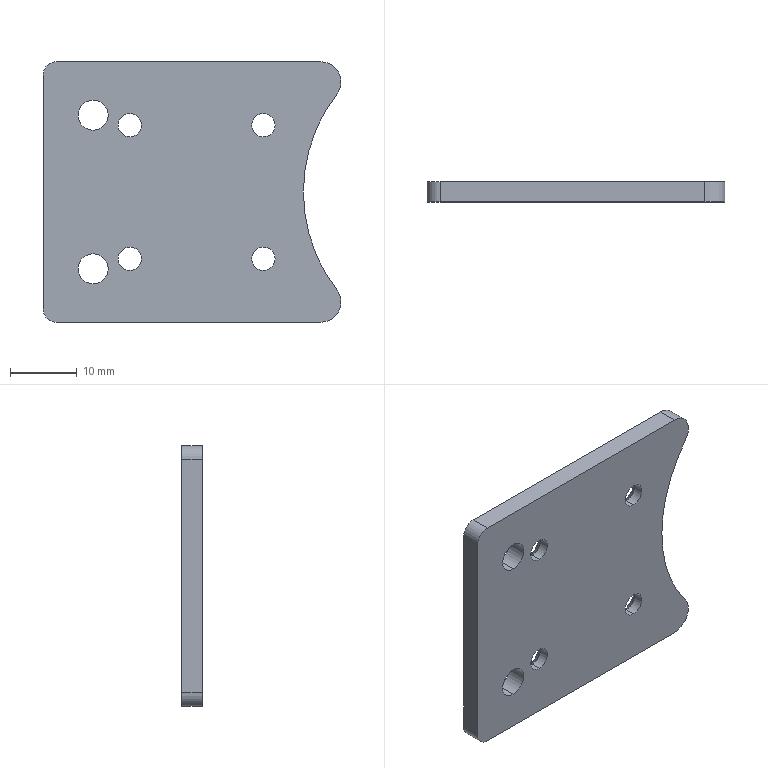CAM job | Mastercam | mm | 1 operations | part box 44.63 x 3 x 39
1. Contour (2D chamfer) | 7 - 4 倒角刀